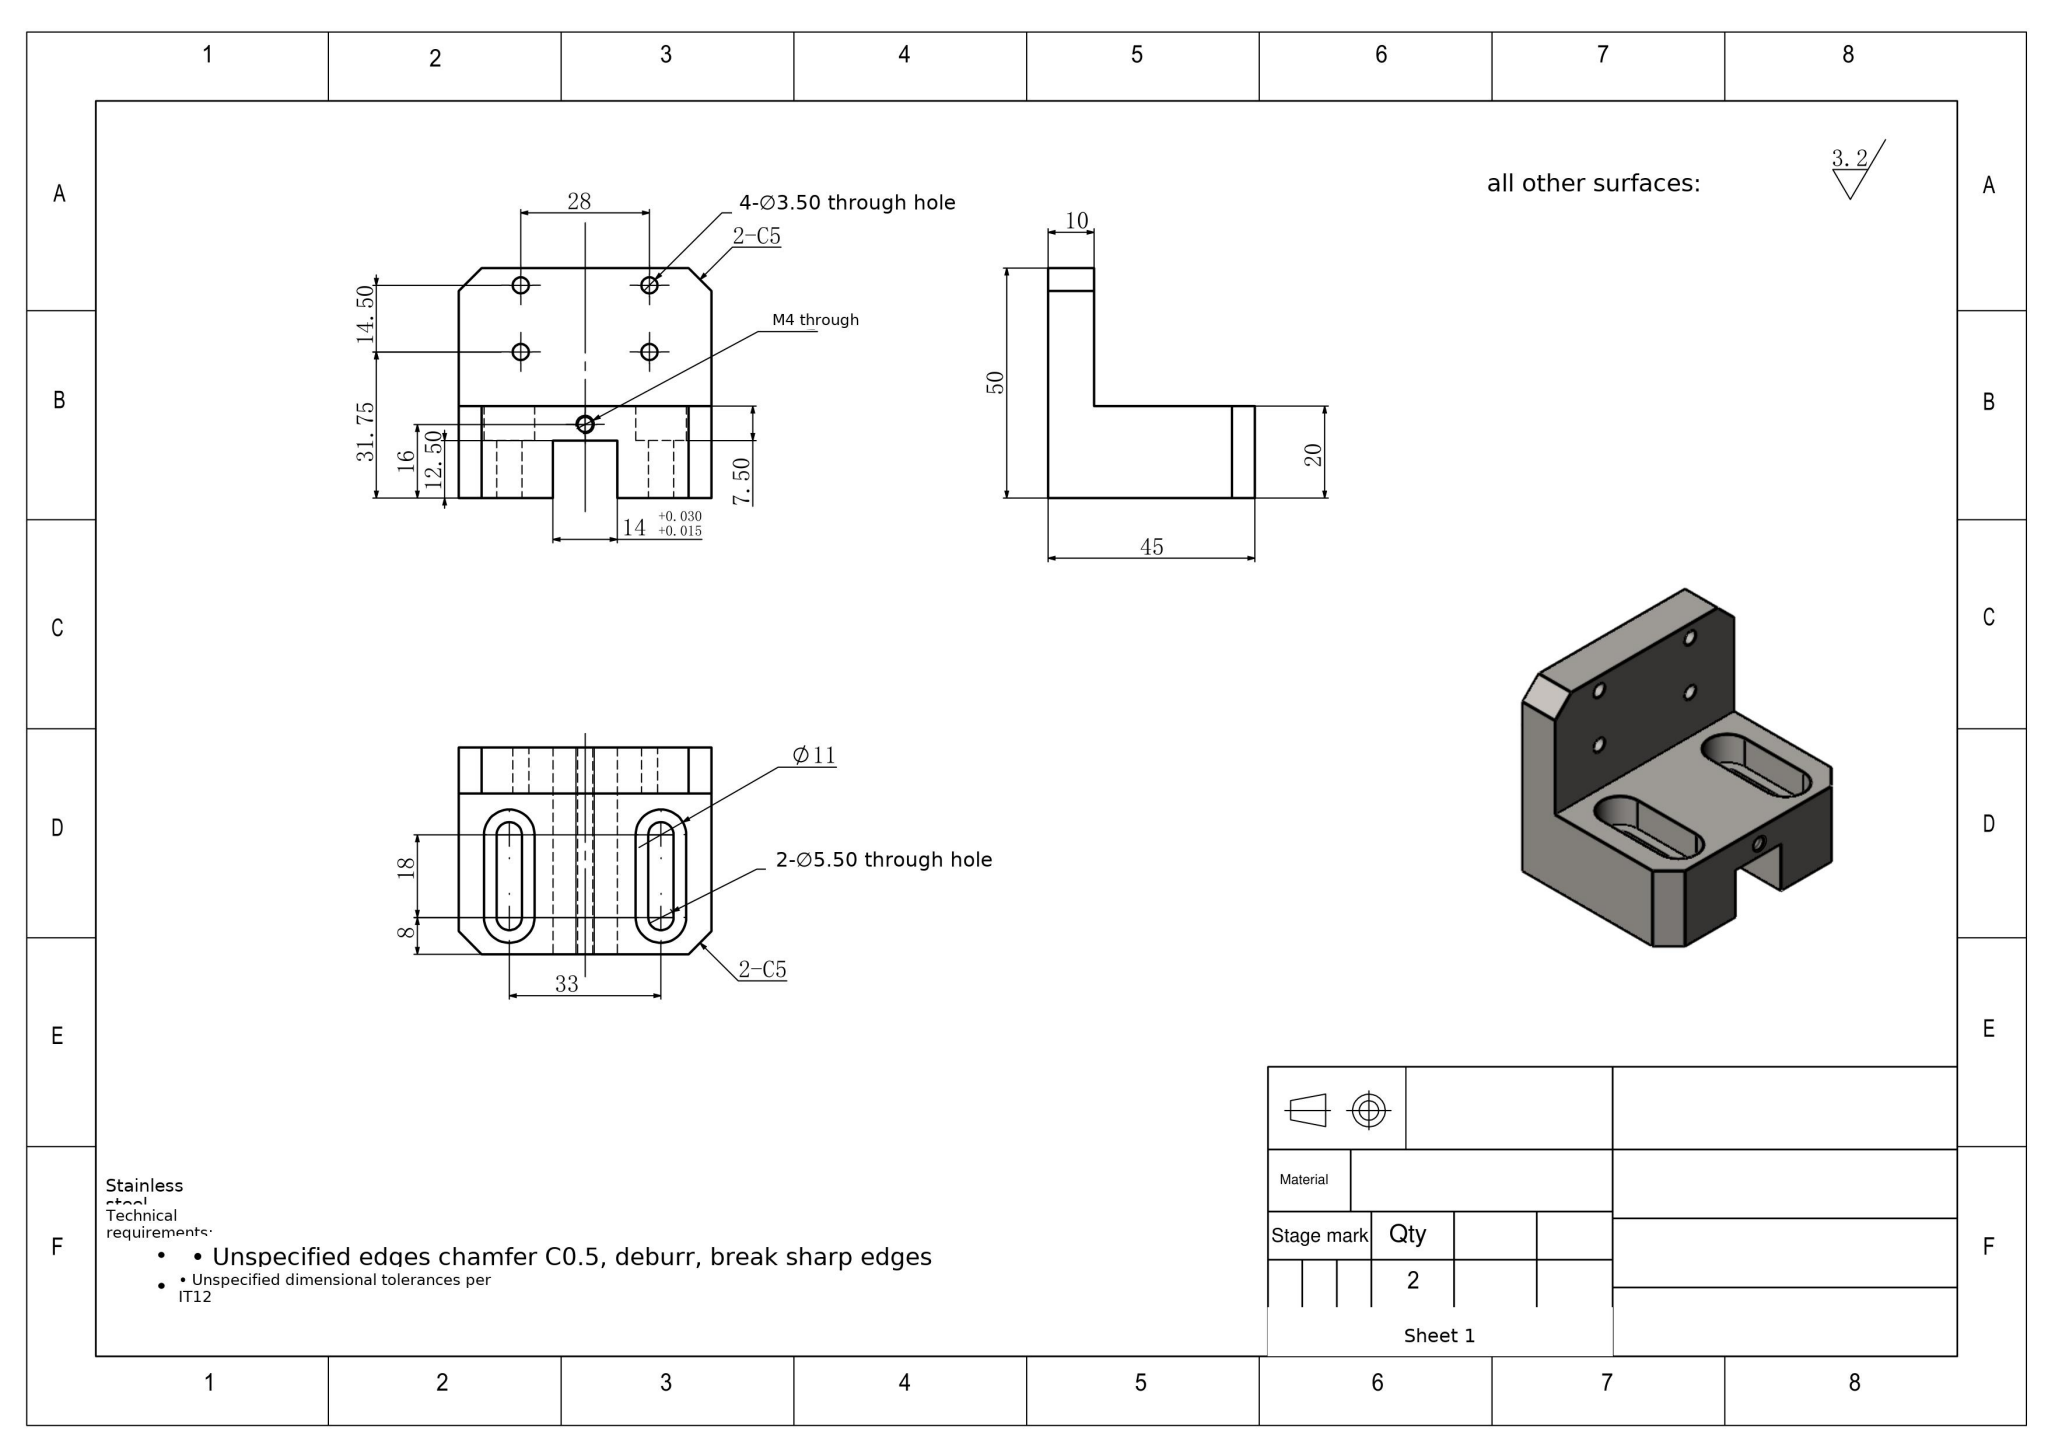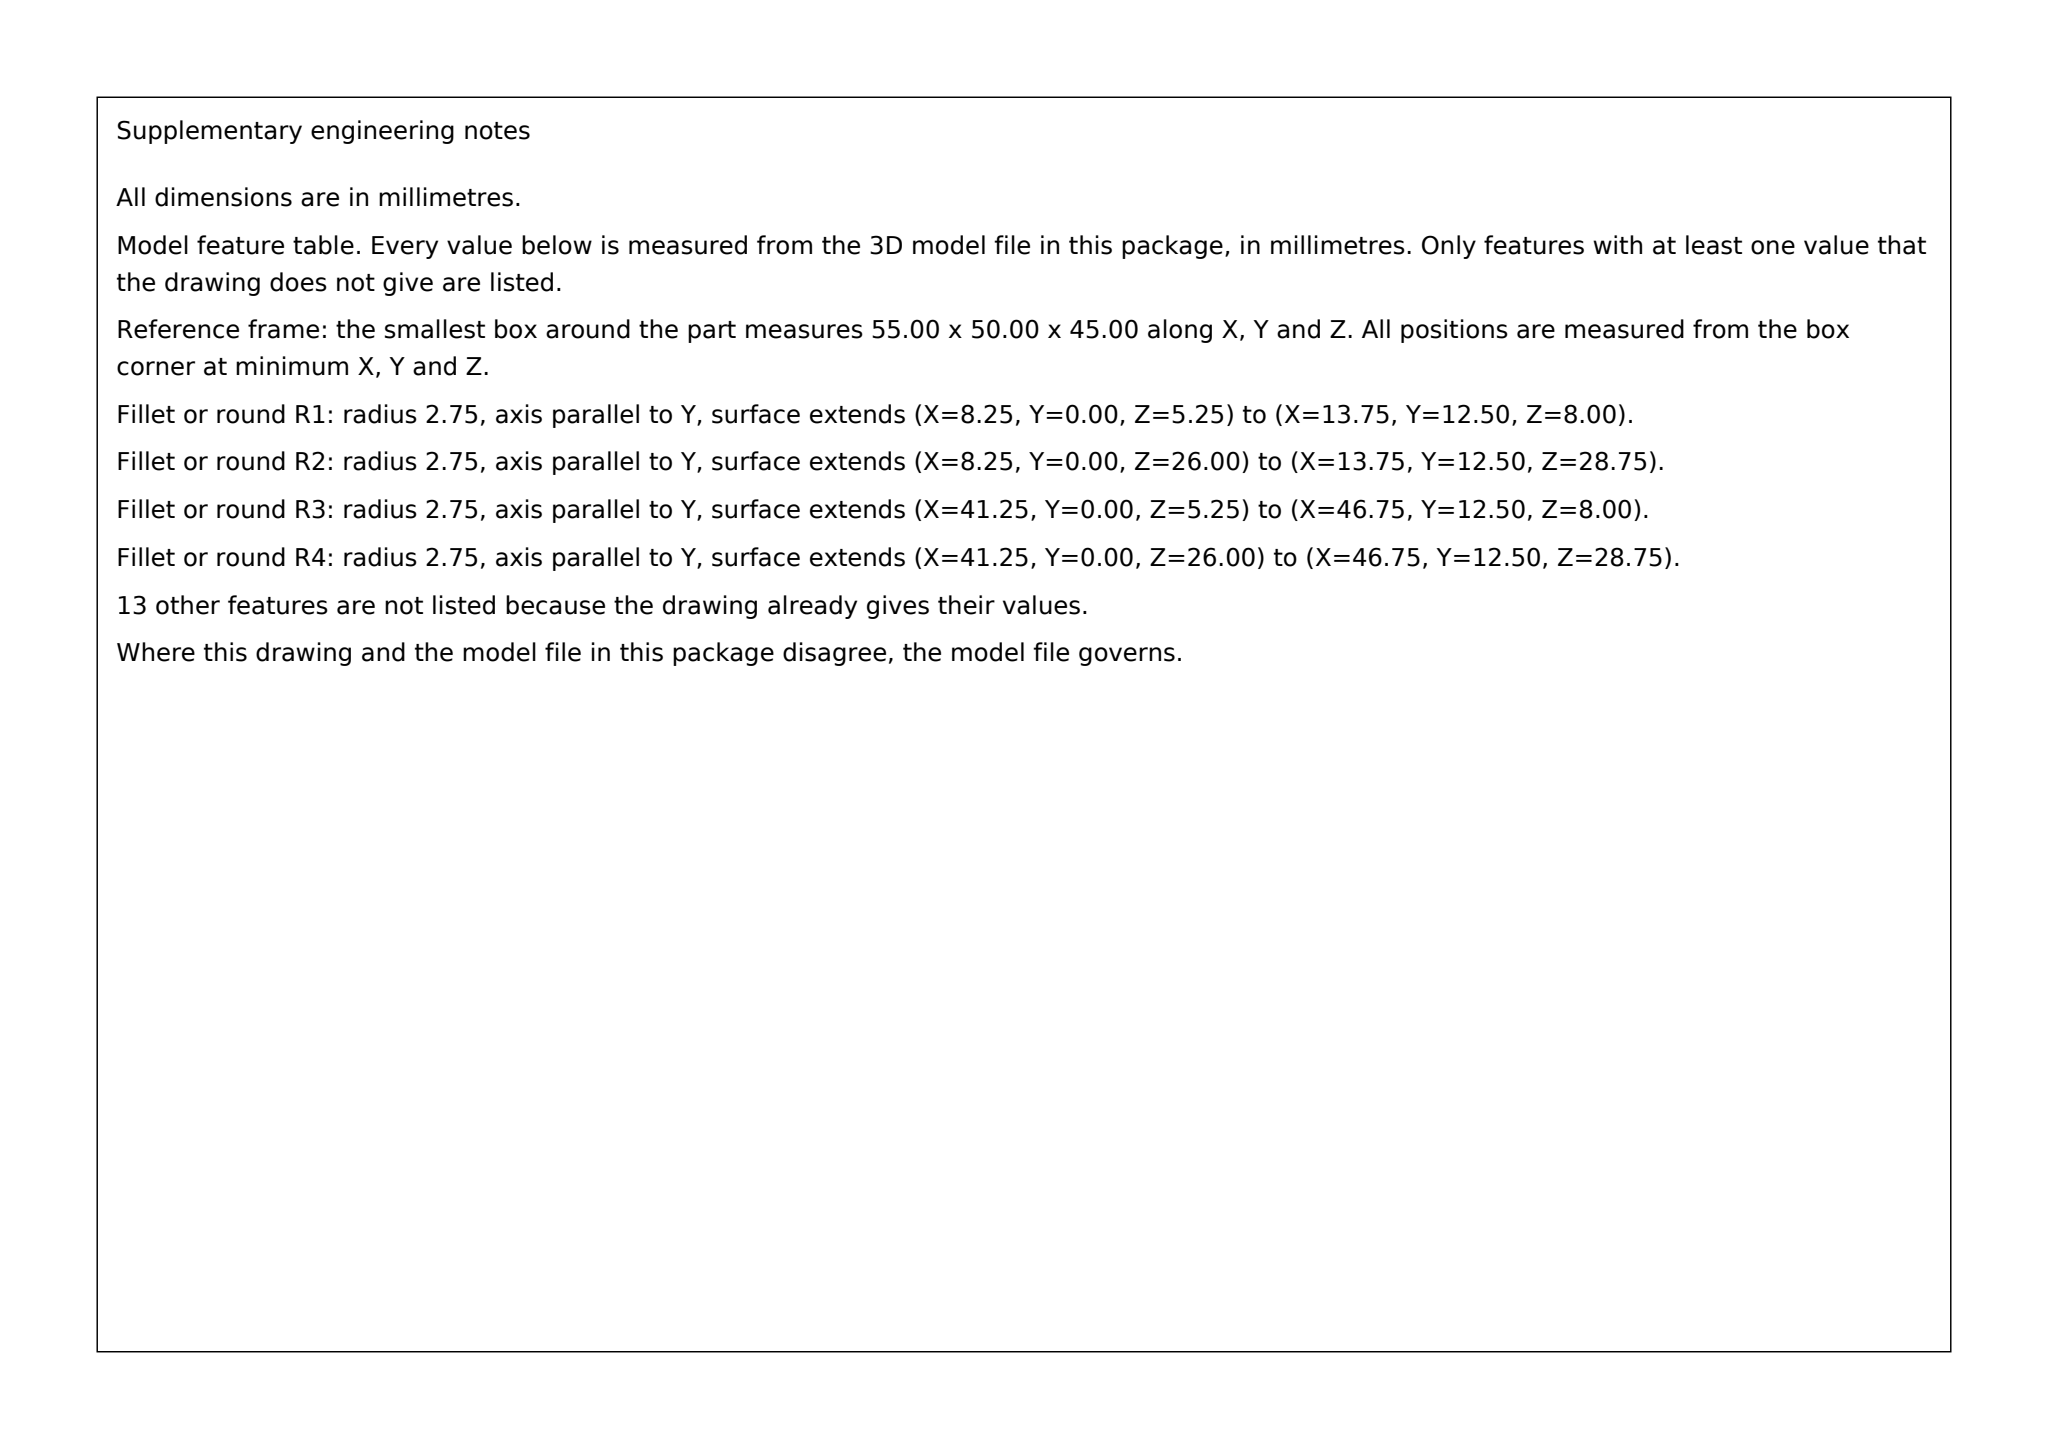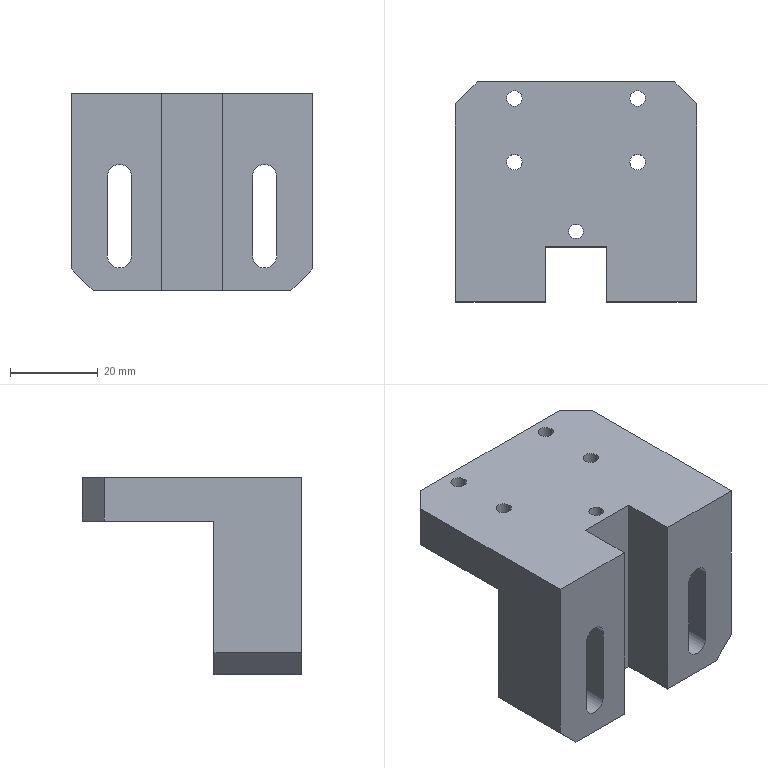Part | SolidWorks | mm | material Stainless steel | 1 solid | 44 faces | box 55 x 50 x 45 mm | volume 49141 mm3 | plane 26 | cylinder 18 | commonest cylinder face diameters 3.5 x8 11 x4 5.5 x4 3.3 x2
build123d program:
from build123d import *

# Parameters (mm, degrees)
BOSS_EXTRUDE1_DEPTH = 45
SKETCH2_R           = 1.75
CUT_EXTRUDE1_DEPTH  = 73.672
SKETCH5_W           = 50.761
SKETCH5_H           = 31.618
CUT_EXTRUDE2_DEPTH  = 87.891
CUT_EXTRUDE3_DEPTH  = 7.5
CUT_EXTRUDE4_DEPTH  = 65.711
M4_TAPPED_HOLE1_D   = 3.3
CHAMFER1_SIZE       = 5


with BuildPart() as part:
    # Sketch1 → Boss-Extrude1 (new body)
    with BuildSketch(Plane.XY):
        Polygon((-27.5, 50), (27.5, 50), (27.5, 0), (7, 0), (7, 12.5), (-7, 12.5), (-7, 0), (-27.5, 0), align=None)
    extrude(amount=BOSS_EXTRUDE1_DEPTH)

    # Sketch2 → Cut-Extrude1 (cut, through all)
    with BuildSketch(Plane.XY.offset(45)):
        with Locations((-14, 46.25)):
            Circle(SKETCH2_R)
        with Locations((-14, 31.75)):
            Circle(SKETCH2_R)
        with Locations((14, 46.25)):
            Circle(SKETCH2_R)
        with Locations((14, 31.75)):
            Circle(SKETCH2_R)
    extrude(amount=-CUT_EXTRUDE1_DEPTH, mode=Mode.SUBTRACT)

    # Sketch5 → Cut-Extrude2 (cut, through all)
    with BuildSketch(Plane.ZY.offset(27.5)):
        with Locations((9.62, 35.809)):
            Rectangle(SKETCH5_W, SKETCH5_H)
    extrude(amount=-CUT_EXTRUDE2_DEPTH, mode=Mode.SUBTRACT)

    # Sketch6 → Cut-Extrude3 (cut)
    with BuildSketch(Plane(origin=(0, 20, 0), x_dir=(1, 0, 0), z_dir=(0, 1, 0))):
        with BuildLine():
            Line((11, -26), (11, -8))
            ThreePointArc((11, -8), (16.5, -2.5), (22, -8))
            Line((22, -8), (22, -26))
            ThreePointArc((22, -26), (16.5, -31.5), (11, -26))
        make_face()
        with BuildLine():
            Line((-11, -26), (-11, -8))
            ThreePointArc((-11, -8), (-16.5, -2.5), (-22, -8))
            Line((-22, -8), (-22, -26))
            ThreePointArc((-22, -26), (-16.5, -31.5), (-11, -26))
        make_face()
    extrude(amount=-CUT_EXTRUDE3_DEPTH, mode=Mode.SUBTRACT)

    # Sketch10 → Cut-Extrude4 (cut, through all)
    with BuildSketch(Plane(origin=(0, 12.5, 0), x_dir=(1, 0, 0), z_dir=(0, 1, 0))):
        with BuildLine():
            Line((19.25, -26), (19.25, -8))
            ThreePointArc((19.25, -8), (16.5, -5.25), (13.75, -8))
            Line((13.75, -8), (13.75, -26))
            ThreePointArc((13.75, -26), (16.5, -28.75), (19.25, -26))
        make_face()
        with BuildLine():
            Line((-13.75, -26), (-13.75, -8))
            ThreePointArc((-13.75, -8), (-16.5, -5.25), (-19.25, -8))
            Line((-19.25, -8), (-19.25, -26))
            ThreePointArc((-19.25, -26), (-16.5, -28.75), (-13.75, -26))
        make_face()
    extrude(amount=-CUT_EXTRUDE4_DEPTH, mode=Mode.SUBTRACT)

    # M4 Tapped Hole1 (through all)
    with Locations(Plane(origin=(0, 0, 0), x_dir=(-1, 0, 0), z_dir=(0, 0, -1))):
        with Locations((0, 16)):
            Hole(M4_TAPPED_HOLE1_D / 2)

    # Chamfer1
    chamfer1_edges = [part.edges().sort_by_distance(p)[0] for p in [
        (-27.5, 50, 40),
        (27.5, 50, 40),
        (-27.5, 10, 0),
        (27.5, 10, 0),
    ]]
    chamfer(chamfer1_edges, length=CHAMFER1_SIZE)


solid = part.part